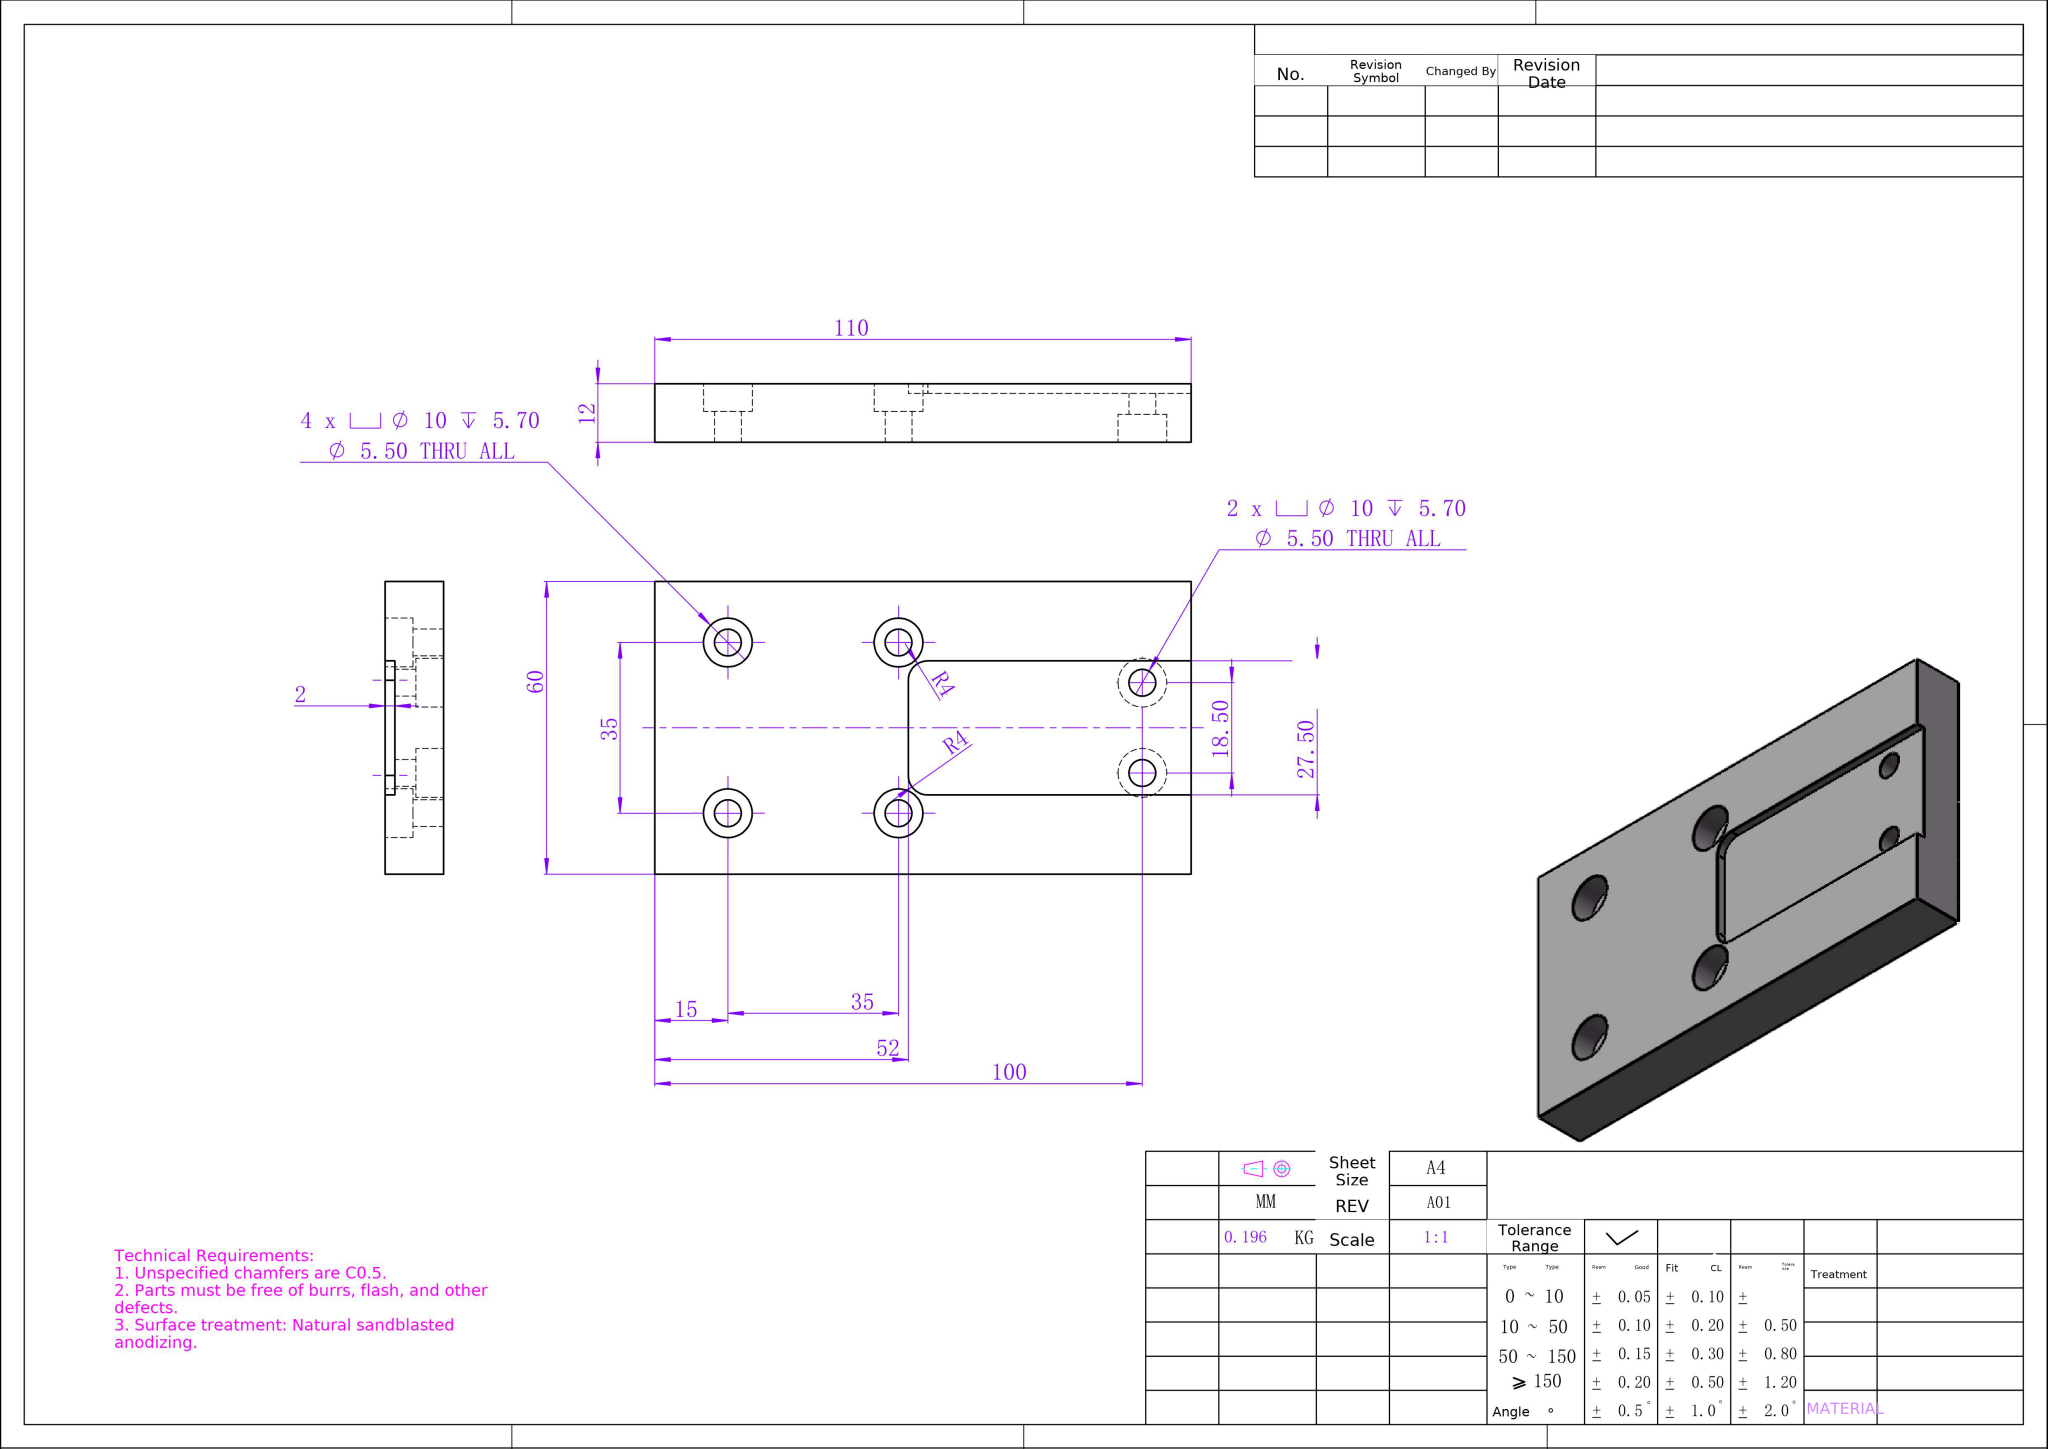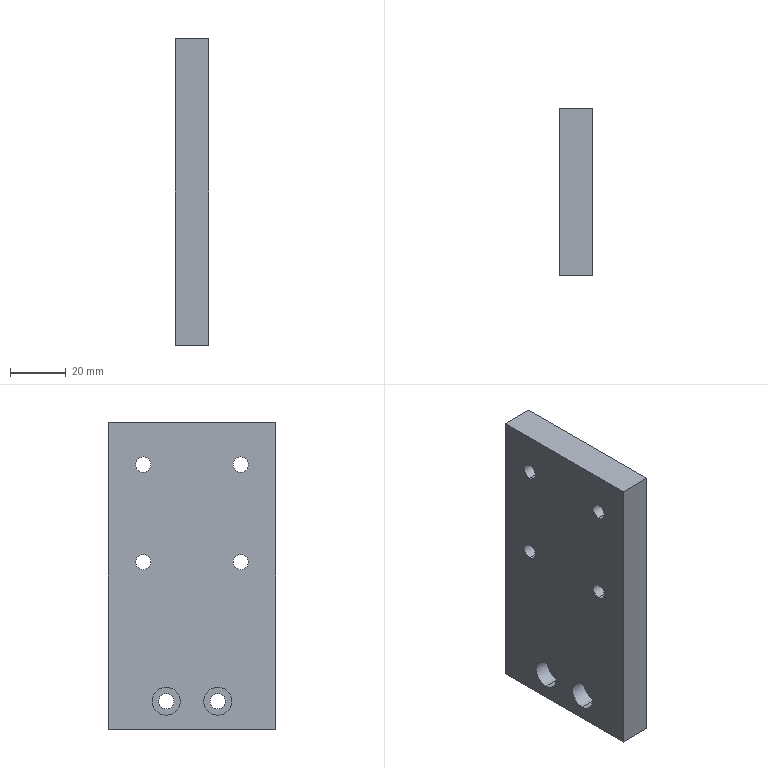Part | NX | mm | 1 solid | 42 faces | box 12 x 60 x 110 mm | volume 72535 mm3 | cylinder 26 | plane 16 | commonest cylinder face diameters 5.5 x12 10 x12 8 x2